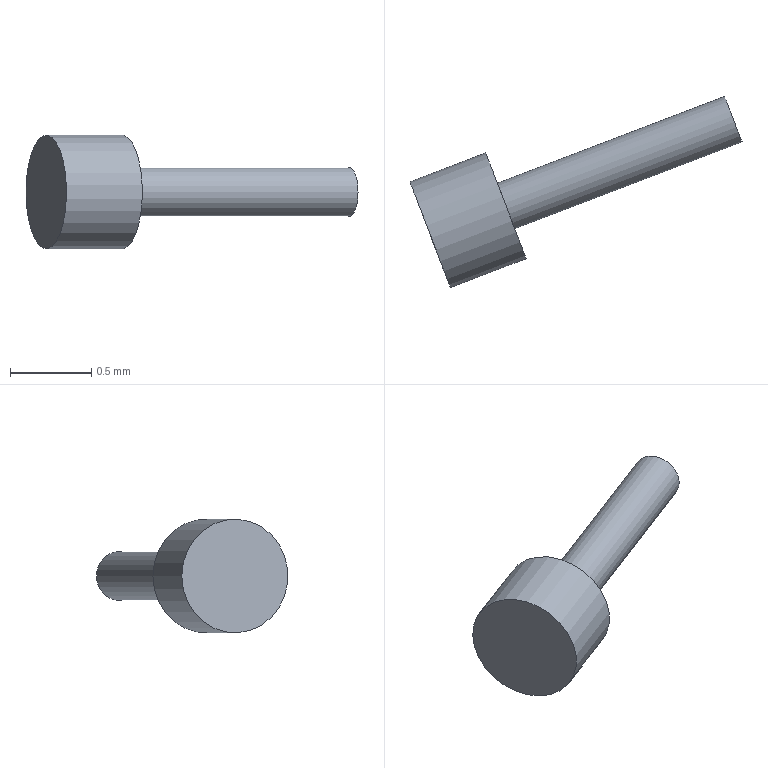Component | NX | BOLT | 1 solid | 5 faces | box 2.05 x 1.18 x 0.7 mm | volume 0 mm3 | plane 3 | cylinder 2 | commonest cylinder face diameters 0.7 x1 0.3 x1
STEP:
#1=CARTESIAN_POINT('',(0.,0.,0.));
#2=DIRECTION('',(0.,0.,1.));
#3=DIRECTION('',(1.,0.,0.));
#4=AXIS2_PLACEMENT_3D('',#1,#2,#3);
#5=CARTESIAN_POINT('',(-1.159,3.036,-4.6));
#6=VERTEX_POINT('',#5);
#7=CARTESIAN_POINT('',(-1.034,2.709,-4.6));
#8=DIRECTION('',(0.9342,0.3566,0.));
#9=DIRECTION('',(-0.3566,0.9342,0.));
#10=AXIS2_PLACEMENT_3D('',#7,#8,#9);
#11=CIRCLE('',#10,0.35);
#12=CARTESIAN_POINT('',(-1.034,2.709,-4.6));
#13=DIRECTION('',(-0.9342,-0.3566,0.));
#14=DIRECTION('',(0.,0.,1.));
#15=AXIS2_PLACEMENT_3D('',#12,#13,#14);
#16=CYLINDRICAL_SURFACE('',#15,0.35);
#17=CARTESIAN_POINT('',(7.854,0.));
#18=DIRECTION('',(-1.,0.));
#19=VECTOR('',#18,1.);
#20=LINE('',#17,#19);
#21=(GEOMETRIC_REPRESENTATION_CONTEXT(2)PARAMETRIC_REPRESENTATION_CONTEXT()REPRESENTATION_CONTEXT('',''));
#22=DEFINITIONAL_REPRESENTATION('',(#20),#21);
#23=PCURVE('',#16,#22);
#24=CARTESIAN_POINT('',(-1.034,2.709,-4.6));
#25=DIRECTION('',(0.9342,0.3566,0.));
#26=DIRECTION('',(0.,0.,-1.));
#27=AXIS2_PLACEMENT_3D('',#24,#25,#26);
#28=PLANE('',#27);
#29=CARTESIAN_POINT('',(0.,0.));
#30=DIRECTION('',(0.,1.));
#31=AXIS2_PLACEMENT_2D('',#29,#30);
#32=CIRCLE('',#31,0.35);
#33=(GEOMETRIC_REPRESENTATION_CONTEXT(2)PARAMETRIC_REPRESENTATION_CONTEXT()REPRESENTATION_CONTEXT('',''));
#34=DEFINITIONAL_REPRESENTATION('',(#32),#33);
#35=PCURVE('',#28,#34);
#36=SURFACE_CURVE('',#11,(#23,#35),.PCURVE_S1.);
#37=EDGE_CURVE('',#6,#6,#36,.T.);
#38=ORIENTED_EDGE('',*,*,#37,.F.);
#39=CARTESIAN_POINT('',(-1.626,2.858,-4.6));
#40=VERTEX_POINT('',#39);
#41=CARTESIAN_POINT('',(-1.159,3.036,-4.6));
#42=CARTESIAN_POINT('',(-1.626,2.858,-4.6));
#43=B_SPLINE_CURVE_WITH_KNOTS('',1,(#41,#42),.UNSPECIFIED.,.F.,.F.,(2,2),(0.,0.5),.PIECEWISE_BEZIER_KNOTS.);
#44=CARTESIAN_POINT('',(7.854,0.));
#45=DIRECTION('',(0.,1.));
#46=VECTOR('',#45,1.);
#47=LINE('',#44,#46);
#48=(GEOMETRIC_REPRESENTATION_CONTEXT(2)PARAMETRIC_REPRESENTATION_CONTEXT()REPRESENTATION_CONTEXT('',''));
#49=DEFINITIONAL_REPRESENTATION('',(#47),#48);
#50=PCURVE('',#16,#49);
#51=CARTESIAN_POINT('',(1.571,0.));
#52=DIRECTION('',(0.,1.));
#53=VECTOR('',#52,1.);
#54=LINE('',#51,#53);
#55=(GEOMETRIC_REPRESENTATION_CONTEXT(2)PARAMETRIC_REPRESENTATION_CONTEXT()REPRESENTATION_CONTEXT('',''));
#56=DEFINITIONAL_REPRESENTATION('',(#54),#55);
#57=PCURVE('',#16,#56);
#58=SEAM_CURVE('',#43,(#50,#57),.PCURVE_S1.);
#59=EDGE_CURVE('',#6,#40,#58,.T.);
#60=ORIENTED_EDGE('',*,*,#59,.T.);
#61=CARTESIAN_POINT('',(-1.501,2.531,-4.6));
#62=DIRECTION('',(0.9342,0.3566,0.));
#63=DIRECTION('',(-0.3566,0.9342,0.));
#64=AXIS2_PLACEMENT_3D('',#61,#62,#63);
#65=CIRCLE('',#64,0.35);
#66=CARTESIAN_POINT('',(7.854,0.5));
#67=DIRECTION('',(-1.,0.));
#68=VECTOR('',#67,1.);
#69=LINE('',#66,#68);
#70=(GEOMETRIC_REPRESENTATION_CONTEXT(2)PARAMETRIC_REPRESENTATION_CONTEXT()REPRESENTATION_CONTEXT('',''));
#71=DEFINITIONAL_REPRESENTATION('',(#69),#70);
#72=PCURVE('',#16,#71);
#73=CARTESIAN_POINT('',(-1.501,2.531,-4.6));
#74=DIRECTION('',(0.9342,0.3566,0.));
#75=DIRECTION('',(0.,0.,-1.));
#76=AXIS2_PLACEMENT_3D('',#73,#74,#75);
#77=PLANE('',#76);
#78=CARTESIAN_POINT('',(0.,0.));
#79=DIRECTION('',(0.,1.));
#80=AXIS2_PLACEMENT_2D('',#78,#79);
#81=CIRCLE('',#80,0.35);
#82=(GEOMETRIC_REPRESENTATION_CONTEXT(2)PARAMETRIC_REPRESENTATION_CONTEXT()REPRESENTATION_CONTEXT('',''));
#83=DEFINITIONAL_REPRESENTATION('',(#81),#82);
#84=PCURVE('',#77,#83);
#85=SURFACE_CURVE('',#65,(#72,#84),.PCURVE_S1.);
#86=EDGE_CURVE('',#40,#40,#85,.T.);
#87=ORIENTED_EDGE('',*,*,#86,.T.);
#88=ORIENTED_EDGE('',*,*,#59,.F.);
#89=EDGE_LOOP('',(#38,#60,#87,#88));
#90=FACE_BOUND('',#89,.T.);
#91=ADVANCED_FACE('',(#90),#16,.T.);
#92=CARTESIAN_POINT('',(-1.088,2.85,-4.6));
#93=VERTEX_POINT('',#92);
#94=CARTESIAN_POINT('',(-1.034,2.709,-4.6));
#95=DIRECTION('',(0.9342,0.3566,0.));
#96=DIRECTION('',(-0.3566,0.9342,0.));
#97=AXIS2_PLACEMENT_3D('',#94,#95,#96);
#98=CIRCLE('',#97,0.15);
#99=CARTESIAN_POINT('',(0.,0.));
#100=DIRECTION('',(0.,1.));
#101=AXIS2_PLACEMENT_2D('',#99,#100);
#102=CIRCLE('',#101,0.15);
#103=(GEOMETRIC_REPRESENTATION_CONTEXT(2)PARAMETRIC_REPRESENTATION_CONTEXT()REPRESENTATION_CONTEXT('',''));
#104=DEFINITIONAL_REPRESENTATION('',(#102),#103);
#105=PCURVE('',#28,#104);
#106=CARTESIAN_POINT('',(0.3671,3.244,-4.6));
#107=DIRECTION('',(-0.9342,-0.3566,0.));
#108=DIRECTION('',(0.,0.,1.));
#109=AXIS2_PLACEMENT_3D('',#106,#107,#108);
#110=CYLINDRICAL_SURFACE('',#109,0.15);
#111=CARTESIAN_POINT('',(7.854,1.5));
#112=DIRECTION('',(-1.,0.));
#113=VECTOR('',#112,1.);
#114=LINE('',#111,#113);
#115=(GEOMETRIC_REPRESENTATION_CONTEXT(2)PARAMETRIC_REPRESENTATION_CONTEXT()REPRESENTATION_CONTEXT('',''));
#116=DEFINITIONAL_REPRESENTATION('',(#114),#115);
#117=PCURVE('',#110,#116);
#118=SURFACE_CURVE('',#98,(#105,#117),.PCURVE_S1.);
#119=EDGE_CURVE('',#93,#93,#118,.T.);
#120=ORIENTED_EDGE('',*,*,#119,.F.);
#121=EDGE_LOOP('',(#120));
#122=FACE_BOUND('',#121,.T.);
#123=ORIENTED_EDGE('',*,*,#37,.T.);
#124=EDGE_LOOP('',(#123));
#125=FACE_BOUND('',#124,.T.);
#126=ADVANCED_FACE('',(#122,#125),#28,.T.);
#127=ORIENTED_EDGE('',*,*,#86,.F.);
#128=EDGE_LOOP('',(#127));
#129=FACE_BOUND('',#128,.T.);
#130=ADVANCED_FACE('',(#129),#77,.F.);
#131=CARTESIAN_POINT('',(0.3136,3.385,-4.6));
#132=VERTEX_POINT('',#131);
#133=CARTESIAN_POINT('',(0.3671,3.244,-4.6));
#134=DIRECTION('',(0.9342,0.3566,0.));
#135=DIRECTION('',(-0.3566,0.9342,0.));
#136=AXIS2_PLACEMENT_3D('',#133,#134,#135);
#137=CIRCLE('',#136,0.15);
#138=CARTESIAN_POINT('',(7.854,0.));
#139=DIRECTION('',(-1.,0.));
#140=VECTOR('',#139,1.);
#141=LINE('',#138,#140);
#142=(GEOMETRIC_REPRESENTATION_CONTEXT(2)PARAMETRIC_REPRESENTATION_CONTEXT()REPRESENTATION_CONTEXT('',''));
#143=DEFINITIONAL_REPRESENTATION('',(#141),#142);
#144=PCURVE('',#110,#143);
#145=CARTESIAN_POINT('',(0.3671,3.244,-4.6));
#146=DIRECTION('',(0.9342,0.3566,0.));
#147=DIRECTION('',(0.,0.,-1.));
#148=AXIS2_PLACEMENT_3D('',#145,#146,#147);
#149=PLANE('',#148);
#150=CARTESIAN_POINT('',(0.,0.));
#151=DIRECTION('',(0.,1.));
#152=AXIS2_PLACEMENT_2D('',#150,#151);
#153=CIRCLE('',#152,0.15);
#154=(GEOMETRIC_REPRESENTATION_CONTEXT(2)PARAMETRIC_REPRESENTATION_CONTEXT()REPRESENTATION_CONTEXT('',''));
#155=DEFINITIONAL_REPRESENTATION('',(#153),#154);
#156=PCURVE('',#149,#155);
#157=SURFACE_CURVE('',#137,(#144,#156),.PCURVE_S1.);
#158=EDGE_CURVE('',#132,#132,#157,.T.);
#159=ORIENTED_EDGE('',*,*,#158,.F.);
#160=CARTESIAN_POINT('',(0.3136,3.385,-4.6));
#161=CARTESIAN_POINT('',(-1.088,2.85,-4.6));
#162=B_SPLINE_CURVE_WITH_KNOTS('',1,(#160,#161),.UNSPECIFIED.,.F.,.F.,(2,2),(0.,1.5),.PIECEWISE_BEZIER_KNOTS.);
#163=CARTESIAN_POINT('',(7.854,0.));
#164=DIRECTION('',(0.,1.));
#165=VECTOR('',#164,1.);
#166=LINE('',#163,#165);
#167=(GEOMETRIC_REPRESENTATION_CONTEXT(2)PARAMETRIC_REPRESENTATION_CONTEXT()REPRESENTATION_CONTEXT('',''));
#168=DEFINITIONAL_REPRESENTATION('',(#166),#167);
#169=PCURVE('',#110,#168);
#170=CARTESIAN_POINT('',(1.571,0.));
#171=DIRECTION('',(0.,1.));
#172=VECTOR('',#171,1.);
#173=LINE('',#170,#172);
#174=(GEOMETRIC_REPRESENTATION_CONTEXT(2)PARAMETRIC_REPRESENTATION_CONTEXT()REPRESENTATION_CONTEXT('',''));
#175=DEFINITIONAL_REPRESENTATION('',(#173),#174);
#176=PCURVE('',#110,#175);
#177=SEAM_CURVE('',#162,(#169,#176),.PCURVE_S1.);
#178=EDGE_CURVE('',#132,#93,#177,.T.);
#179=ORIENTED_EDGE('',*,*,#178,.T.);
#180=ORIENTED_EDGE('',*,*,#119,.T.);
#181=ORIENTED_EDGE('',*,*,#178,.F.);
#182=EDGE_LOOP('',(#159,#179,#180,#181));
#183=FACE_BOUND('',#182,.T.);
#184=ADVANCED_FACE('',(#183),#110,.T.);
#185=ORIENTED_EDGE('',*,*,#158,.T.);
#186=EDGE_LOOP('',(#185));
#187=FACE_BOUND('',#186,.T.);
#188=ADVANCED_FACE('',(#187),#149,.T.);
#189=CLOSED_SHELL('',(#91,#126,#130,#184,#188));
#190=MANIFOLD_SOLID_BREP('',#189);
#191=(LENGTH_UNIT()NAMED_UNIT(*)SI_UNIT(.MILLI.,.METRE.));
#192=UNCERTAINTY_MEASURE_WITH_UNIT(LENGTH_MEASURE(0.00001),#191,'','');
#193=(NAMED_UNIT(*)PLANE_ANGLE_UNIT()SI_UNIT($,.RADIAN.));
#194=(NAMED_UNIT(*)SI_UNIT($,.STERADIAN.)SOLID_ANGLE_UNIT());
#195=(GEOMETRIC_REPRESENTATION_CONTEXT(3)GLOBAL_UNCERTAINTY_ASSIGNED_CONTEXT((#192))GLOBAL_UNIT_ASSIGNED_CONTEXT((#191,#193,#194))REPRESENTATION_CONTEXT('',''));
#196=ADVANCED_BREP_SHAPE_REPRESENTATION('',(#4,#190),#195);